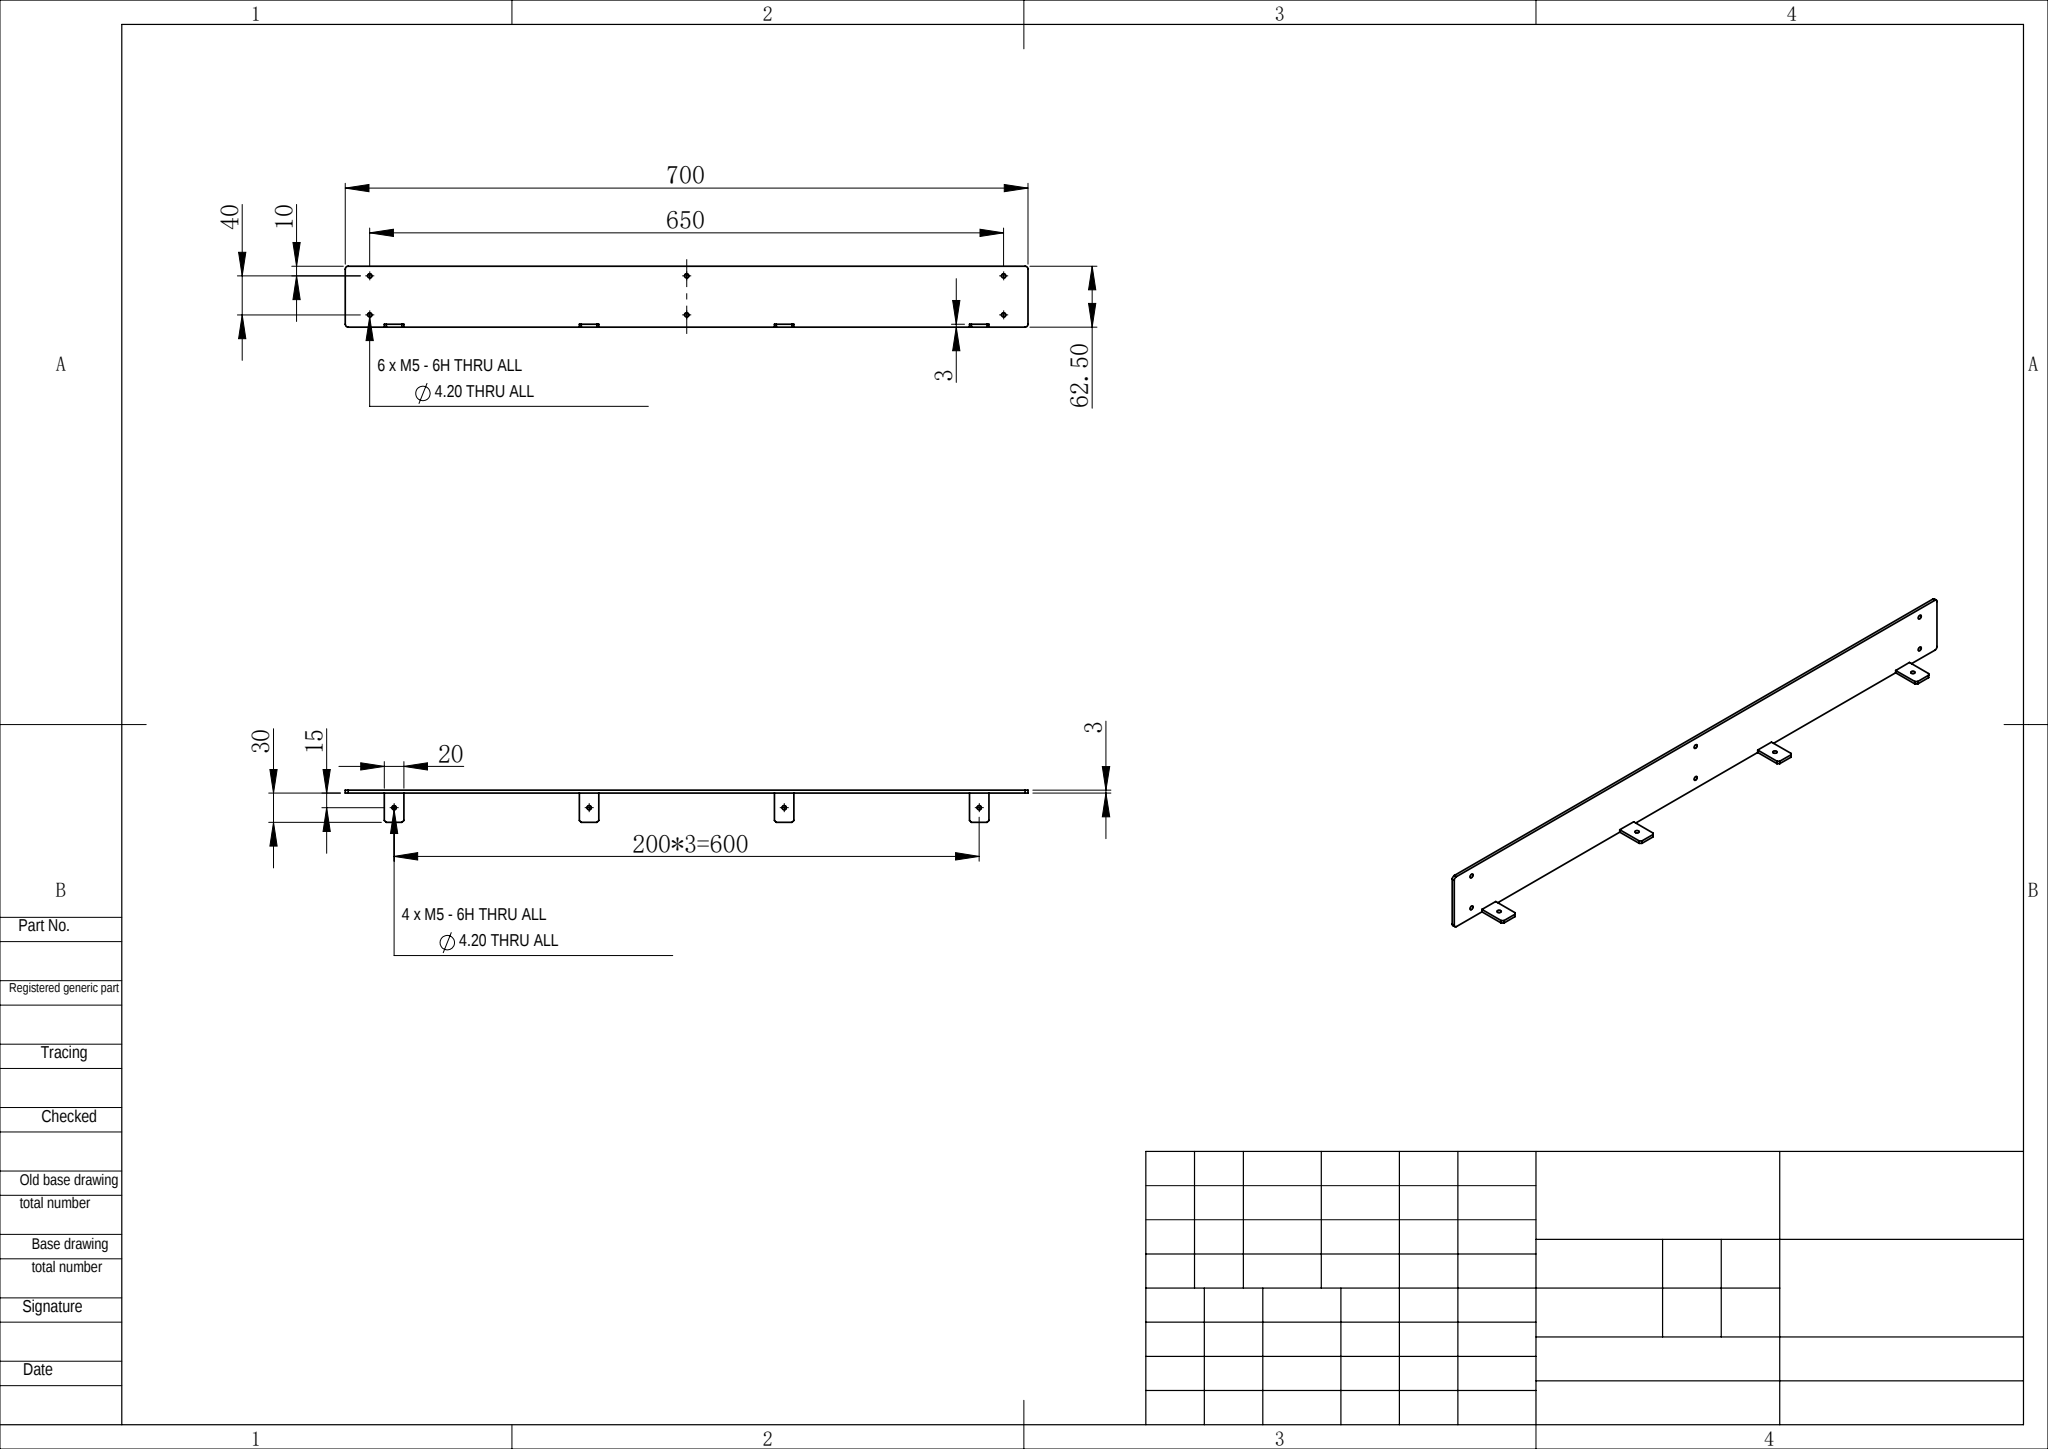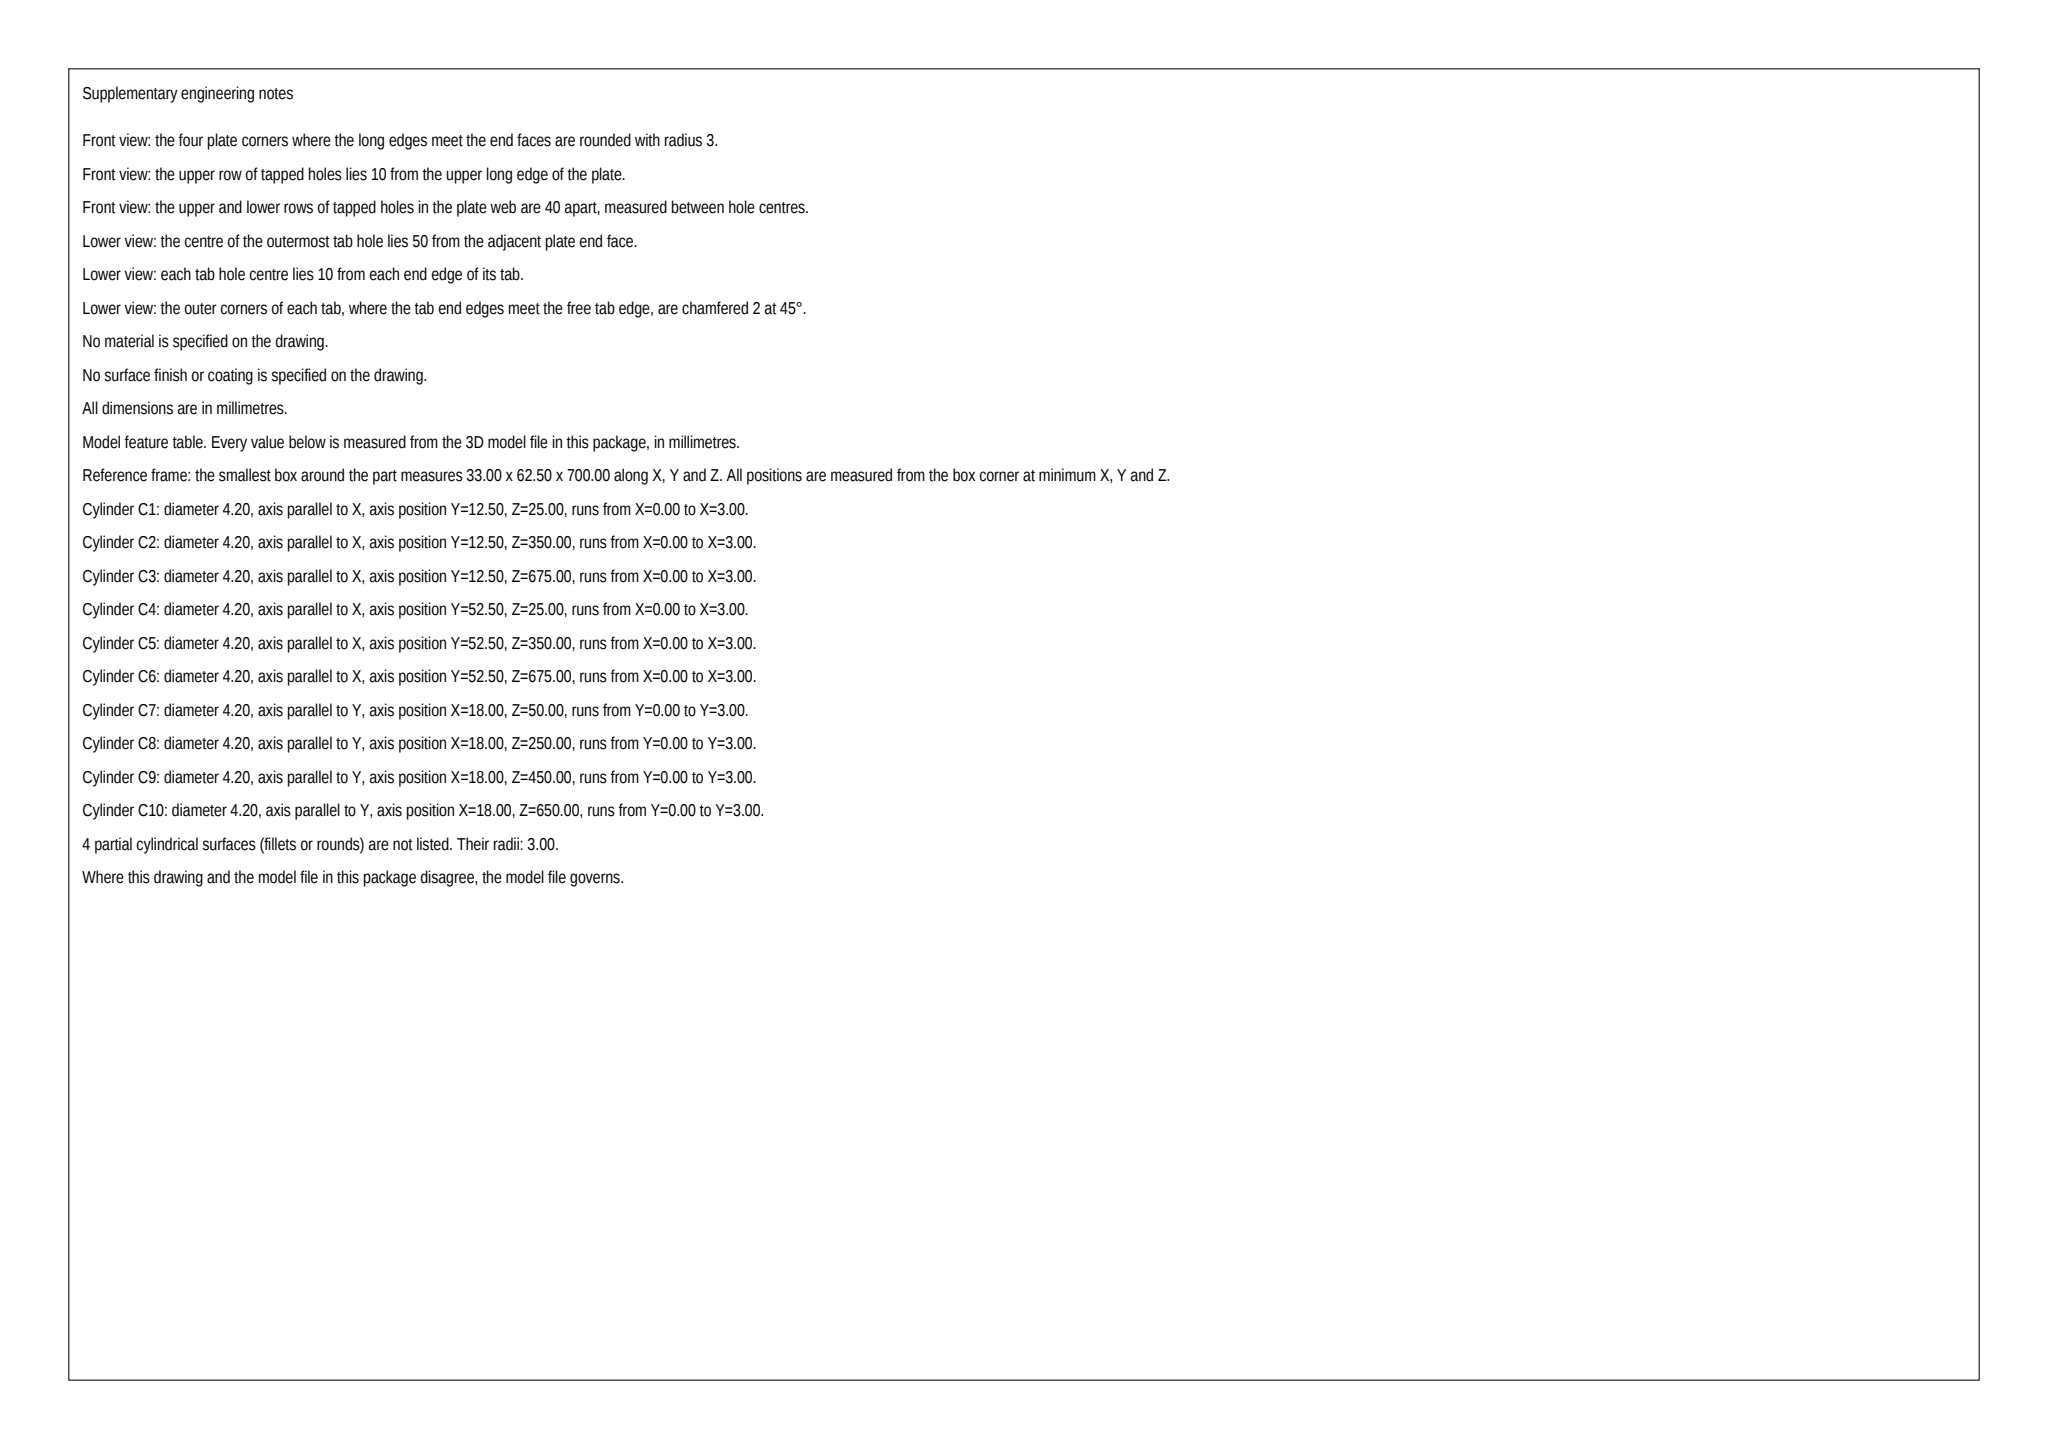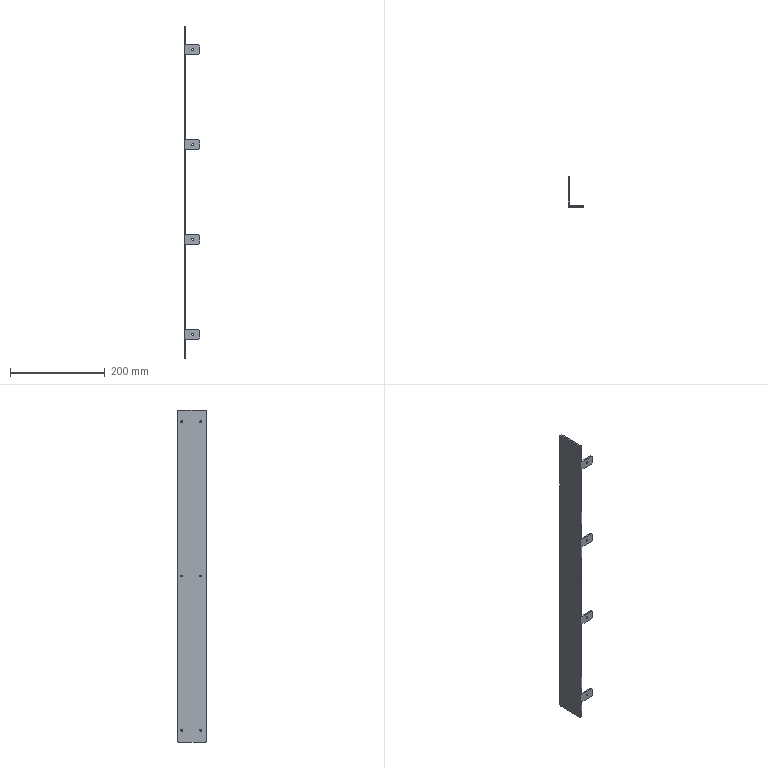Part | SolidWorks | mm | 1 solid | 54 faces | box 33 x 62.5 x 700 mm | volume 137963 mm3 | plane 30 | cylinder 24 | commonest cylinder face diameters 4.2 x20 6 x4